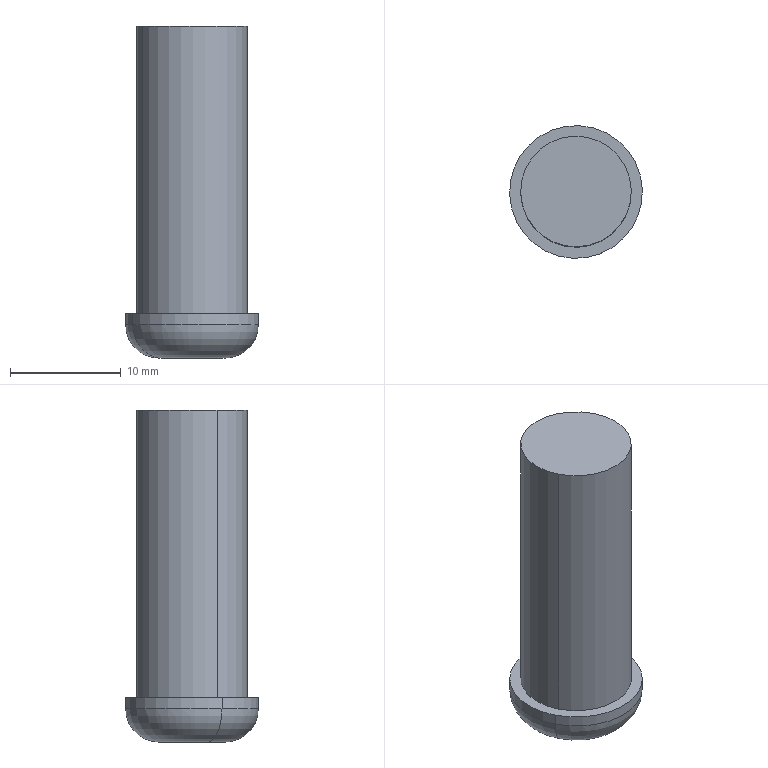Component | SolidWorks | FixedPin26mm-1 | 1 solid | 9 faces | box 12 x 12 x 30 mm | volume 2430 mm3 | cylinder 4 | plane 3 | torus 2 | commonest cylinder face diameters 12 x2 10 x2
build123d program:
from build123d import *

# Parameters (mm, degrees)
SKETCH1_R           = 5
BOSS_EXTRUDE1_DEPTH = 26
SKETCH2_R           = 6
BOSS_EXTRUDE2_DEPTH = 4
FILLET1_R           = 3


with BuildPart() as part:
    # Sketch1 → Boss-Extrude1 (new body)
    with BuildSketch(Plane.XY):
        with Locations(Location((0, 0, 0), (0, 0, 180))):
            Circle(SKETCH1_R)
    extrude(amount=BOSS_EXTRUDE1_DEPTH)

    # Sketch2 → Boss-Extrude2 (add)
    with BuildSketch(Plane.XY.offset(26)):
        Circle(SKETCH2_R)
    extrude(amount=BOSS_EXTRUDE2_DEPTH)

    # Fillet1
    fillet1_edges = [part.edges().sort_by_distance(p)[0] for p in [
        (-6, 0, 30),
    ]]
    fillet(fillet1_edges, radius=FILLET1_R)


solid = part.part

# Placed as in the assembly
solid = solid.moved(Location((65.366, -4.894, 142.846), (180, 0, 0)))
STEP:
#1=COLOUR_RGB('',0.7922,0.8196,0.9333);
#2=FILL_AREA_STYLE_COLOUR('',#1);
#3=FILL_AREA_STYLE('',(#2));
#4=SURFACE_STYLE_FILL_AREA(#3);
#5=SURFACE_SIDE_STYLE('',(#4));
#6=SURFACE_STYLE_USAGE(.BOTH.,#5);
#7=PRESENTATION_STYLE_ASSIGNMENT((#6));
#8=CARTESIAN_POINT('',(2.784,-0.08594,4.561));
#9=VERTEX_POINT('',#8);
#10=CARTESIAN_POINT('',(2.363,-0.2994,4.561));
#11=VERTEX_POINT('',#10);
#12=CARTESIAN_POINT('',(2.573,-0.1927,4.561));
#13=DIRECTION('',(0.,0.,1.));
#14=DIRECTION('',(-0.8921,-0.4519,0.));
#15=AXIS2_PLACEMENT_3D('',#12,#13,#14);
#16=CIRCLE('',#15,0.2362);
#17=EDGE_CURVE('',#9,#11,#16,.T.);
#18=ORIENTED_EDGE('',*,*,#17,.F.);
#19=CARTESIAN_POINT('',(2.679,-0.1393,4.443));
#20=VERTEX_POINT('',#19);
#21=CARTESIAN_POINT('',(2.679,-0.1393,4.561));
#22=DIRECTION('',(-0.4519,0.8921,0.));
#23=DIRECTION('',(-0.8921,-0.4519,0.));
#24=AXIS2_PLACEMENT_3D('',#21,#22,#23);
#25=CIRCLE('',#24,0.1181);
#26=EDGE_CURVE('',#9,#20,#25,.T.);
#27=ORIENTED_EDGE('',*,*,#26,.T.);
#28=CARTESIAN_POINT('',(2.468,-0.2461,4.443));
#29=VERTEX_POINT('',#28);
#30=CARTESIAN_POINT('',(2.573,-0.1927,4.443));
#31=DIRECTION('',(0.,0.,-1.));
#32=DIRECTION('',(-0.8921,-0.4519,0.));
#33=AXIS2_PLACEMENT_3D('',#30,#31,#32);
#34=CIRCLE('',#33,0.1181);
#35=EDGE_CURVE('',#29,#20,#34,.T.);
#36=ORIENTED_EDGE('',*,*,#35,.F.);
#37=CARTESIAN_POINT('',(2.468,-0.2461,4.561));
#38=DIRECTION('',(0.4519,-0.8921,0.));
#39=DIRECTION('',(0.8921,0.4519,0.));
#40=AXIS2_PLACEMENT_3D('',#37,#38,#39);
#41=CIRCLE('',#40,0.1181);
#42=EDGE_CURVE('',#11,#29,#41,.T.);
#43=ORIENTED_EDGE('',*,*,#42,.F.);
#44=EDGE_LOOP('',(#18,#27,#36,#43));
#45=FACE_OUTER_BOUND('',#44,.T.);
#46=CARTESIAN_POINT('',(2.573,-0.1927,4.561));
#47=DIRECTION('',(0.,0.,-1.));
#48=DIRECTION('',(-0.8921,-0.4519,0.));
#49=AXIS2_PLACEMENT_3D('',#46,#47,#48);
#50=TOROIDAL_SURFACE('',#49,0.1181,0.1181);
#51=ADVANCED_FACE('',(#45),#50,.T.);
#52=ORIENTED_EDGE('',*,*,#17,.T.);
#53=CARTESIAN_POINT('',(2.363,-0.2994,4.6));
#54=VERTEX_POINT('',#53);
#55=CARTESIAN_POINT('',(2.363,-0.2994,4.443));
#56=DIRECTION('',(0.,0.,1.));
#57=VECTOR('',#56,39.37);
#58=LINE('',#55,#57);
#59=EDGE_CURVE('',#11,#54,#58,.T.);
#60=ORIENTED_EDGE('',*,*,#59,.T.);
#61=CARTESIAN_POINT('',(2.784,-0.08594,4.6));
#62=VERTEX_POINT('',#61);
#63=CARTESIAN_POINT('',(2.573,-0.1927,4.6));
#64=DIRECTION('',(0.,0.,-1.));
#65=DIRECTION('',(-0.8921,-0.4519,0.));
#66=AXIS2_PLACEMENT_3D('',#63,#64,#65);
#67=CIRCLE('',#66,0.2362);
#68=EDGE_CURVE('',#54,#62,#67,.T.);
#69=ORIENTED_EDGE('',*,*,#68,.T.);
#70=CARTESIAN_POINT('',(2.784,-0.08594,4.443));
#71=DIRECTION('',(0.,0.,1.));
#72=VECTOR('',#71,39.37);
#73=LINE('',#70,#72);
#74=EDGE_CURVE('',#9,#62,#73,.T.);
#75=ORIENTED_EDGE('',*,*,#74,.F.);
#76=EDGE_LOOP('',(#52,#60,#69,#75));
#77=FACE_OUTER_BOUND('',#76,.T.);
#78=CARTESIAN_POINT('',(2.573,-0.1927,4.443));
#79=DIRECTION('',(0.,0.,1.));
#80=DIRECTION('',(0.8921,0.4519,0.));
#81=AXIS2_PLACEMENT_3D('',#78,#79,#80);
#82=CYLINDRICAL_SURFACE('',#81,0.2362);
#83=ADVANCED_FACE('',(#77),#82,.T.);
#84=CARTESIAN_POINT('',(2.398,-0.2816,4.6));
#85=VERTEX_POINT('',#84);
#86=CARTESIAN_POINT('',(2.749,-0.1037,4.6));
#87=VERTEX_POINT('',#86);
#88=CARTESIAN_POINT('',(2.573,-0.1927,4.6));
#89=DIRECTION('',(0.,0.,-1.));
#90=DIRECTION('',(-0.8921,-0.4519,0.));
#91=AXIS2_PLACEMENT_3D('',#88,#89,#90);
#92=CIRCLE('',#91,0.1969);
#93=EDGE_CURVE('',#85,#87,#92,.T.);
#94=ORIENTED_EDGE('',*,*,#93,.F.);
#95=CARTESIAN_POINT('',(2.398,-0.2816,5.624));
#96=VERTEX_POINT('',#95);
#97=CARTESIAN_POINT('',(2.398,-0.2816,4.6));
#98=DIRECTION('',(0.,0.,1.));
#99=VECTOR('',#98,39.37);
#100=LINE('',#97,#99);
#101=EDGE_CURVE('',#85,#96,#100,.T.);
#102=ORIENTED_EDGE('',*,*,#101,.T.);
#103=CARTESIAN_POINT('',(2.749,-0.1037,5.624));
#104=VERTEX_POINT('',#103);
#105=CARTESIAN_POINT('',(2.573,-0.1927,5.624));
#106=DIRECTION('',(0.,0.,-1.));
#107=DIRECTION('',(-0.8921,-0.4519,0.));
#108=AXIS2_PLACEMENT_3D('',#105,#106,#107);
#109=CIRCLE('',#108,0.1969);
#110=EDGE_CURVE('',#96,#104,#109,.T.);
#111=ORIENTED_EDGE('',*,*,#110,.T.);
#112=CARTESIAN_POINT('',(2.749,-0.1037,4.6));
#113=DIRECTION('',(0.,0.,1.));
#114=VECTOR('',#113,39.37);
#115=LINE('',#112,#114);
#116=EDGE_CURVE('',#87,#104,#115,.T.);
#117=ORIENTED_EDGE('',*,*,#116,.F.);
#118=EDGE_LOOP('',(#94,#102,#111,#117));
#119=FACE_OUTER_BOUND('',#118,.T.);
#120=CARTESIAN_POINT('',(2.573,-0.1927,4.6));
#121=DIRECTION('',(0.,0.,1.));
#122=DIRECTION('',(0.8921,0.4519,0.));
#123=AXIS2_PLACEMENT_3D('',#120,#121,#122);
#124=CYLINDRICAL_SURFACE('',#123,0.1969);
#125=ADVANCED_FACE('',(#119),#124,.T.);
#126=ORIENTED_EDGE('',*,*,#101,.F.);
#127=CARTESIAN_POINT('',(2.573,-0.1927,4.6));
#128=DIRECTION('',(0.,0.,-1.));
#129=DIRECTION('',(-0.8921,-0.4519,0.));
#130=AXIS2_PLACEMENT_3D('',#127,#128,#129);
#131=CIRCLE('',#130,0.1969);
#132=EDGE_CURVE('',#87,#85,#131,.T.);
#133=ORIENTED_EDGE('',*,*,#132,.F.);
#134=ORIENTED_EDGE('',*,*,#116,.T.);
#135=CARTESIAN_POINT('',(2.573,-0.1927,5.624));
#136=DIRECTION('',(0.,0.,-1.));
#137=DIRECTION('',(-0.8921,-0.4519,0.));
#138=AXIS2_PLACEMENT_3D('',#135,#136,#137);
#139=CIRCLE('',#138,0.1969);
#140=EDGE_CURVE('',#104,#96,#139,.T.);
#141=ORIENTED_EDGE('',*,*,#140,.T.);
#142=EDGE_LOOP('',(#126,#133,#134,#141));
#143=FACE_OUTER_BOUND('',#142,.T.);
#144=CARTESIAN_POINT('',(2.573,-0.1927,4.6));
#145=DIRECTION('',(0.,0.,1.));
#146=DIRECTION('',(0.8921,0.4519,0.));
#147=AXIS2_PLACEMENT_3D('',#144,#145,#146);
#148=CYLINDRICAL_SURFACE('',#147,0.1969);
#149=ADVANCED_FACE('',(#143),#148,.T.);
#150=ORIENTED_EDGE('',*,*,#140,.F.);
#151=ORIENTED_EDGE('',*,*,#110,.F.);
#152=EDGE_LOOP('',(#150,#151));
#153=FACE_OUTER_BOUND('',#152,.T.);
#154=CARTESIAN_POINT('',(2.573,-0.1927,5.624));
#155=DIRECTION('',(0.,0.,-1.));
#156=DIRECTION('',(-0.8921,-0.4519,0.));
#157=AXIS2_PLACEMENT_3D('',#154,#155,#156);
#158=PLANE('',#157);
#159=ADVANCED_FACE('',(#153),#158,.F.);
#160=ORIENTED_EDGE('',*,*,#59,.F.);
#161=CARTESIAN_POINT('',(2.573,-0.1927,4.561));
#162=DIRECTION('',(0.,0.,1.));
#163=DIRECTION('',(-0.8921,-0.4519,0.));
#164=AXIS2_PLACEMENT_3D('',#161,#162,#163);
#165=CIRCLE('',#164,0.2362);
#166=EDGE_CURVE('',#11,#9,#165,.T.);
#167=ORIENTED_EDGE('',*,*,#166,.T.);
#168=ORIENTED_EDGE('',*,*,#74,.T.);
#169=CARTESIAN_POINT('',(2.573,-0.1927,4.6));
#170=DIRECTION('',(0.,0.,-1.));
#171=DIRECTION('',(-0.8921,-0.4519,0.));
#172=AXIS2_PLACEMENT_3D('',#169,#170,#171);
#173=CIRCLE('',#172,0.2362);
#174=EDGE_CURVE('',#62,#54,#173,.T.);
#175=ORIENTED_EDGE('',*,*,#174,.T.);
#176=EDGE_LOOP('',(#160,#167,#168,#175));
#177=FACE_OUTER_BOUND('',#176,.T.);
#178=CARTESIAN_POINT('',(2.573,-0.1927,4.443));
#179=DIRECTION('',(0.,0.,1.));
#180=DIRECTION('',(0.8921,0.4519,0.));
#181=AXIS2_PLACEMENT_3D('',#178,#179,#180);
#182=CYLINDRICAL_SURFACE('',#181,0.2362);
#183=ADVANCED_FACE('',(#177),#182,.T.);
#184=ORIENTED_EDGE('',*,*,#35,.T.);
#185=CARTESIAN_POINT('',(2.573,-0.1927,4.443));
#186=DIRECTION('',(0.,0.,-1.));
#187=DIRECTION('',(-0.8921,-0.4519,0.));
#188=AXIS2_PLACEMENT_3D('',#185,#186,#187);
#189=CIRCLE('',#188,0.1181);
#190=EDGE_CURVE('',#20,#29,#189,.T.);
#191=ORIENTED_EDGE('',*,*,#190,.T.);
#192=EDGE_LOOP('',(#184,#191));
#193=FACE_OUTER_BOUND('',#192,.T.);
#194=CARTESIAN_POINT('',(2.573,-0.1927,4.443));
#195=DIRECTION('',(0.,0.,-1.));
#196=DIRECTION('',(-0.8921,-0.4519,0.));
#197=AXIS2_PLACEMENT_3D('',#194,#195,#196);
#198=PLANE('',#197);
#199=ADVANCED_FACE('',(#193),#198,.T.);
#200=ORIENTED_EDGE('',*,*,#132,.T.);
#201=ORIENTED_EDGE('',*,*,#93,.T.);
#202=EDGE_LOOP('',(#200,#201));
#203=FACE_BOUND('',#202,.T.);
#204=ORIENTED_EDGE('',*,*,#174,.F.);
#205=ORIENTED_EDGE('',*,*,#68,.F.);
#206=EDGE_LOOP('',(#204,#205));
#207=FACE_OUTER_BOUND('',#206,.T.);
#208=CARTESIAN_POINT('',(2.573,-0.1927,4.6));
#209=DIRECTION('',(0.,0.,-1.));
#210=DIRECTION('',(-0.8921,-0.4519,0.));
#211=AXIS2_PLACEMENT_3D('',#208,#209,#210);
#212=PLANE('',#211);
#213=ADVANCED_FACE('',(#203,#207),#212,.F.);
#214=ORIENTED_EDGE('',*,*,#26,.F.);
#215=ORIENTED_EDGE('',*,*,#166,.F.);
#216=ORIENTED_EDGE('',*,*,#42,.T.);
#217=ORIENTED_EDGE('',*,*,#190,.F.);
#218=EDGE_LOOP('',(#214,#215,#216,#217));
#219=FACE_OUTER_BOUND('',#218,.T.);
#220=CARTESIAN_POINT('',(2.573,-0.1927,4.561));
#221=DIRECTION('',(0.,0.,-1.));
#222=DIRECTION('',(-0.8921,-0.4519,0.));
#223=AXIS2_PLACEMENT_3D('',#220,#221,#222);
#224=TOROIDAL_SURFACE('',#223,0.1181,0.1181);
#225=ADVANCED_FACE('',(#219),#224,.T.);
#226=CLOSED_SHELL('',(#51,#83,#125,#149,#159,#183,#199,#213,#225));
#227=MANIFOLD_SOLID_BREP('',#226);
#228=STYLED_ITEM('',(#7),#227);
#229=(LENGTH_UNIT()NAMED_UNIT(*)SI_UNIT($,.METRE.));
#230=LENGTH_MEASURE_WITH_UNIT(LENGTH_MEASURE(0.0254),#229);
#231=DIMENSIONAL_EXPONENTS(1.,0.,0.,0.,0.,0.,0.);
#232=(CONVERSION_BASED_UNIT('',#230)LENGTH_UNIT()NAMED_UNIT(#231));
#233=UNCERTAINTY_MEASURE_WITH_UNIT(LENGTH_MEASURE(0.00001),#232,'','');
#234=(NAMED_UNIT(*)PLANE_ANGLE_UNIT()SI_UNIT($,.RADIAN.));
#235=(NAMED_UNIT(*)SI_UNIT($,.STERADIAN.)SOLID_ANGLE_UNIT());
#236=(GEOMETRIC_REPRESENTATION_CONTEXT(3)GLOBAL_UNCERTAINTY_ASSIGNED_CONTEXT((#233))GLOBAL_UNIT_ASSIGNED_CONTEXT((#232,#234,#235))REPRESENTATION_CONTEXT('',''));
#237=MECHANICAL_DESIGN_GEOMETRIC_PRESENTATION_REPRESENTATION('',(#228),#236);
#238=CARTESIAN_POINT('',(0.,0.,0.));
#239=DIRECTION('',(0.,0.,1.));
#240=DIRECTION('',(1.,0.,0.));
#241=AXIS2_PLACEMENT_3D('',#238,#239,#240);
#242=(LENGTH_UNIT()NAMED_UNIT(*)SI_UNIT($,.METRE.));
#243=LENGTH_MEASURE_WITH_UNIT(LENGTH_MEASURE(0.0254),#242);
#244=DIMENSIONAL_EXPONENTS(1.,0.,0.,0.,0.,0.,0.);
#245=(CONVERSION_BASED_UNIT('',#243)LENGTH_UNIT()NAMED_UNIT(#244));
#246=UNCERTAINTY_MEASURE_WITH_UNIT(LENGTH_MEASURE(0.00001),#245,'','');
#247=(NAMED_UNIT(*)PLANE_ANGLE_UNIT()SI_UNIT($,.RADIAN.));
#248=(NAMED_UNIT(*)SI_UNIT($,.STERADIAN.)SOLID_ANGLE_UNIT());
#249=(GEOMETRIC_REPRESENTATION_CONTEXT(3)GLOBAL_UNCERTAINTY_ASSIGNED_CONTEXT((#246))GLOBAL_UNIT_ASSIGNED_CONTEXT((#245,#247,#248))REPRESENTATION_CONTEXT('',''));
#250=ADVANCED_BREP_SHAPE_REPRESENTATION('',(#227,#241),#249);
#251=PRESENTATION_LAYER_ASSIGNMENT('','',(#228));